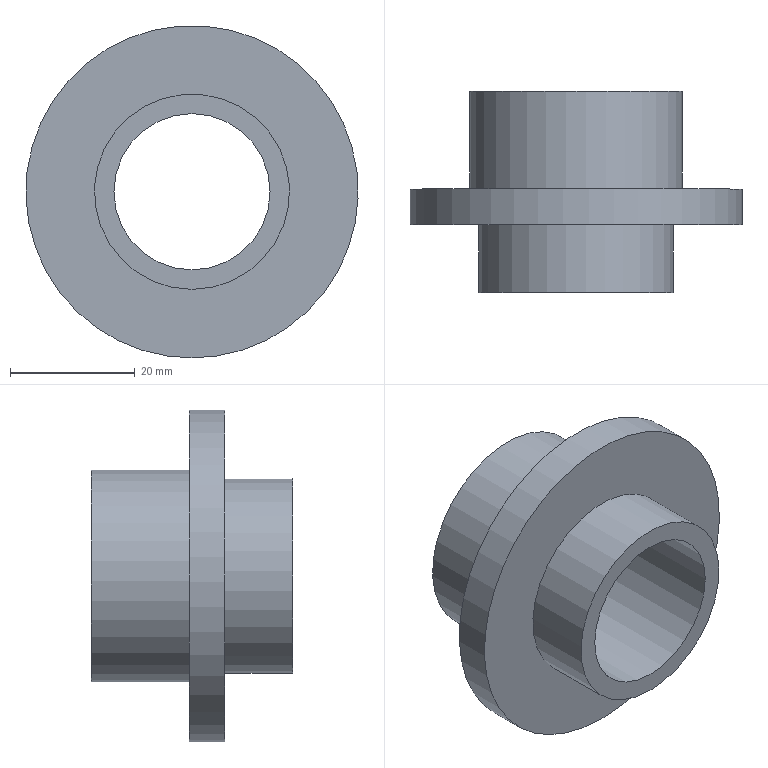Component | NX | SPRING_SLEEVE_1 | 1 solid | 8 faces | box 53.17 x 32.19 x 53.17 mm | volume 19347 mm3 | cylinder 4 | plane 4 | commonest cylinder face diameters 53.169 x1 31.237 x1 25 x1 34 x1
STEP:
#1=CARTESIAN_POINT('',(0.,0.,0.));
#2=DIRECTION('',(0.,0.,1.));
#3=DIRECTION('',(1.,0.,0.));
#4=AXIS2_PLACEMENT_3D('',#1,#2,#3);
#5=CARTESIAN_POINT('',(0.,0.,-26.584));
#6=VERTEX_POINT('',#5);
#7=CARTESIAN_POINT('',(0.,0.,0.));
#8=DIRECTION('',(0.,-1.,0.));
#9=DIRECTION('',(0.,0.,-1.));
#10=AXIS2_PLACEMENT_3D('',#7,#8,#9);
#11=CIRCLE('',#10,26.584);
#12=CARTESIAN_POINT('',(0.,0.,0.));
#13=DIRECTION('',(0.,-1.,0.));
#14=DIRECTION('',(0.,0.,-1.));
#15=AXIS2_PLACEMENT_3D('',#12,#13,#14);
#16=CYLINDRICAL_SURFACE('',#15,26.584);
#17=CARTESIAN_POINT('',(0.,-0.));
#18=DIRECTION('',(1.,0.));
#19=VECTOR('',#18,1.);
#20=LINE('',#17,#19);
#21=(GEOMETRIC_REPRESENTATION_CONTEXT(2)PARAMETRIC_REPRESENTATION_CONTEXT()REPRESENTATION_CONTEXT('',''));
#22=DEFINITIONAL_REPRESENTATION('',(#20),#21);
#23=PCURVE('',#16,#22);
#24=CARTESIAN_POINT('',(-26.584,0.,0.));
#25=DIRECTION('',(0.,1.,0.));
#26=DIRECTION('',(0.,0.,1.));
#27=AXIS2_PLACEMENT_3D('',#24,#25,#26);
#28=PLANE('',#27);
#29=CARTESIAN_POINT('',(-26.584,26.584));
#30=CARTESIAN_POINT('',(-26.584,72.63));
#31=CARTESIAN_POINT('',(13.292,49.607));
#32=CARTESIAN_POINT('',(53.169,26.584));
#33=CARTESIAN_POINT('',(13.292,3.562));
#34=CARTESIAN_POINT('',(-26.584,-19.461));
#35=CARTESIAN_POINT('',(-26.584,26.584));
#36=(BOUNDED_CURVE()B_SPLINE_CURVE(2,(#29,#30,#31,#32,#33,#34,#35),.UNSPECIFIED.,.T.,.F.)B_SPLINE_CURVE_WITH_KNOTS((1,2,2,2,2,1),(-2.094,0.,2.094,4.189,6.283,8.378),.UNSPECIFIED.)CURVE()GEOMETRIC_REPRESENTATION_ITEM()RATIONAL_B_SPLINE_CURVE((1.,0.5,1.,0.5,1.,0.5,1.))REPRESENTATION_ITEM(''));
#37=(GEOMETRIC_REPRESENTATION_CONTEXT(2)PARAMETRIC_REPRESENTATION_CONTEXT()REPRESENTATION_CONTEXT('',''));
#38=DEFINITIONAL_REPRESENTATION('',(#36),#37);
#39=PCURVE('',#28,#38);
#40=SURFACE_CURVE('',#11,(#23,#39),.PCURVE_S1.);
#41=EDGE_CURVE('',#6,#6,#40,.T.);
#42=ORIENTED_EDGE('',*,*,#41,.F.);
#43=CARTESIAN_POINT('',(0.,5.684,-26.584));
#44=VERTEX_POINT('',#43);
#45=CARTESIAN_POINT('',(-0.,5.684,-26.584));
#46=CARTESIAN_POINT('',(-0.,0.,-26.584));
#47=B_SPLINE_CURVE_WITH_KNOTS('',1,(#45,#46),.UNSPECIFIED.,.F.,.F.,(2,2),(-5.684,-0.),.PIECEWISE_BEZIER_KNOTS.);
#48=CARTESIAN_POINT('',(0.,0.));
#49=DIRECTION('',(0.,1.));
#50=VECTOR('',#49,1.);
#51=LINE('',#48,#50);
#52=(GEOMETRIC_REPRESENTATION_CONTEXT(2)PARAMETRIC_REPRESENTATION_CONTEXT()REPRESENTATION_CONTEXT('',''));
#53=DEFINITIONAL_REPRESENTATION('',(#51),#52);
#54=PCURVE('',#16,#53);
#55=CARTESIAN_POINT('',(6.283,0.));
#56=DIRECTION('',(0.,1.));
#57=VECTOR('',#56,1.);
#58=LINE('',#55,#57);
#59=(GEOMETRIC_REPRESENTATION_CONTEXT(2)PARAMETRIC_REPRESENTATION_CONTEXT()REPRESENTATION_CONTEXT('',''));
#60=DEFINITIONAL_REPRESENTATION('',(#58),#59);
#61=PCURVE('',#16,#60);
#62=SEAM_CURVE('',#47,(#54,#61),.PCURVE_S1.);
#63=EDGE_CURVE('',#44,#6,#62,.T.);
#64=ORIENTED_EDGE('',*,*,#63,.F.);
#65=CARTESIAN_POINT('',(0.,5.684,0.));
#66=DIRECTION('',(0.,-1.,0.));
#67=DIRECTION('',(0.,0.,-1.));
#68=AXIS2_PLACEMENT_3D('',#65,#66,#67);
#69=CIRCLE('',#68,26.584);
#70=CARTESIAN_POINT('',(0.,-5.684));
#71=DIRECTION('',(1.,0.));
#72=VECTOR('',#71,1.);
#73=LINE('',#70,#72);
#74=(GEOMETRIC_REPRESENTATION_CONTEXT(2)PARAMETRIC_REPRESENTATION_CONTEXT()REPRESENTATION_CONTEXT('',''));
#75=DEFINITIONAL_REPRESENTATION('',(#73),#74);
#76=PCURVE('',#16,#75);
#77=CARTESIAN_POINT('',(-17.456,5.684,0.));
#78=DIRECTION('',(0.,-1.,0.));
#79=DIRECTION('',(0.,0.,-1.));
#80=AXIS2_PLACEMENT_3D('',#77,#78,#79);
#81=PLANE('',#80);
#82=CARTESIAN_POINT('',(0.,17.456));
#83=DIRECTION('',(1.,0.));
#84=AXIS2_PLACEMENT_2D('',#82,#83);
#85=CIRCLE('',#84,26.584);
#86=(GEOMETRIC_REPRESENTATION_CONTEXT(2)PARAMETRIC_REPRESENTATION_CONTEXT()REPRESENTATION_CONTEXT('',''));
#87=DEFINITIONAL_REPRESENTATION('',(#85),#86);
#88=PCURVE('',#81,#87);
#89=SURFACE_CURVE('',#69,(#76,#88),.PCURVE_S1.);
#90=EDGE_CURVE('',#44,#44,#89,.T.);
#91=ORIENTED_EDGE('',*,*,#90,.T.);
#92=ORIENTED_EDGE('',*,*,#63,.T.);
#93=EDGE_LOOP('',(#42,#64,#91,#92));
#94=FACE_BOUND('',#93,.T.);
#95=ADVANCED_FACE('',(#94),#16,.T.);
#96=CARTESIAN_POINT('',(0.,0.,-15.619));
#97=VERTEX_POINT('',#96);
#98=CARTESIAN_POINT('',(0.,0.,0.));
#99=DIRECTION('',(0.,-1.,0.));
#100=DIRECTION('',(0.,0.,-1.));
#101=AXIS2_PLACEMENT_3D('',#98,#99,#100);
#102=CIRCLE('',#101,15.619);
#103=CARTESIAN_POINT('',(-15.619,26.584));
#104=CARTESIAN_POINT('',(-15.619,53.637));
#105=CARTESIAN_POINT('',(7.809,40.111));
#106=CARTESIAN_POINT('',(31.237,26.584));
#107=CARTESIAN_POINT('',(7.809,13.058));
#108=CARTESIAN_POINT('',(-15.619,-0.4679));
#109=CARTESIAN_POINT('',(-15.619,26.584));
#110=(BOUNDED_CURVE()B_SPLINE_CURVE(2,(#103,#104,#105,#106,#107,#108,#109),.UNSPECIFIED.,.T.,.F.)B_SPLINE_CURVE_WITH_KNOTS((1,2,2,2,2,1),(-2.094,0.,2.094,4.189,6.283,8.378),.UNSPECIFIED.)CURVE()GEOMETRIC_REPRESENTATION_ITEM()RATIONAL_B_SPLINE_CURVE((1.,0.5,1.,0.5,1.,0.5,1.))REPRESENTATION_ITEM(''));
#111=(GEOMETRIC_REPRESENTATION_CONTEXT(2)PARAMETRIC_REPRESENTATION_CONTEXT()REPRESENTATION_CONTEXT('',''));
#112=DEFINITIONAL_REPRESENTATION('',(#110),#111);
#113=PCURVE('',#28,#112);
#114=CARTESIAN_POINT('',(0.,0.,0.));
#115=DIRECTION('',(0.,-1.,0.));
#116=DIRECTION('',(0.,0.,-1.));
#117=AXIS2_PLACEMENT_3D('',#114,#115,#116);
#118=CYLINDRICAL_SURFACE('',#117,15.619);
#119=CARTESIAN_POINT('',(0.,0.));
#120=DIRECTION('',(1.,0.));
#121=VECTOR('',#120,1.);
#122=LINE('',#119,#121);
#123=(GEOMETRIC_REPRESENTATION_CONTEXT(2)PARAMETRIC_REPRESENTATION_CONTEXT()REPRESENTATION_CONTEXT('',''));
#124=DEFINITIONAL_REPRESENTATION('',(#122),#123);
#125=PCURVE('',#118,#124);
#126=SURFACE_CURVE('',#102,(#113,#125),.PCURVE_S1.);
#127=EDGE_CURVE('',#97,#97,#126,.T.);
#128=ORIENTED_EDGE('',*,*,#127,.F.);
#129=EDGE_LOOP('',(#128));
#130=FACE_BOUND('',#129,.T.);
#131=ORIENTED_EDGE('',*,*,#41,.T.);
#132=EDGE_LOOP('',(#131));
#133=FACE_BOUND('',#132,.T.);
#134=ADVANCED_FACE('',(#130,#133),#28,.F.);
#135=CARTESIAN_POINT('',(0.,-10.877,-15.619));
#136=VERTEX_POINT('',#135);
#137=CARTESIAN_POINT('',(0.,-10.877,0.));
#138=DIRECTION('',(0.,-1.,0.));
#139=DIRECTION('',(0.,0.,-1.));
#140=AXIS2_PLACEMENT_3D('',#137,#138,#139);
#141=CIRCLE('',#140,15.619);
#142=CARTESIAN_POINT('',(0.,10.877));
#143=DIRECTION('',(1.,0.));
#144=VECTOR('',#143,1.);
#145=LINE('',#142,#144);
#146=(GEOMETRIC_REPRESENTATION_CONTEXT(2)PARAMETRIC_REPRESENTATION_CONTEXT()REPRESENTATION_CONTEXT('',''));
#147=DEFINITIONAL_REPRESENTATION('',(#145),#146);
#148=PCURVE('',#118,#147);
#149=CARTESIAN_POINT('',(-15.619,-10.877,0.));
#150=DIRECTION('',(0.,1.,0.));
#151=DIRECTION('',(0.,0.,1.));
#152=AXIS2_PLACEMENT_3D('',#149,#150,#151);
#153=PLANE('',#152);
#154=CARTESIAN_POINT('',(-15.619,15.619));
#155=CARTESIAN_POINT('',(-15.619,42.671));
#156=CARTESIAN_POINT('',(7.809,29.145));
#157=CARTESIAN_POINT('',(31.237,15.619));
#158=CARTESIAN_POINT('',(7.809,2.093));
#159=CARTESIAN_POINT('',(-15.619,-11.434));
#160=CARTESIAN_POINT('',(-15.619,15.619));
#161=(BOUNDED_CURVE()B_SPLINE_CURVE(2,(#154,#155,#156,#157,#158,#159,#160),.UNSPECIFIED.,.T.,.F.)B_SPLINE_CURVE_WITH_KNOTS((1,2,2,2,2,1),(-2.094,0.,2.094,4.189,6.283,8.378),.UNSPECIFIED.)CURVE()GEOMETRIC_REPRESENTATION_ITEM()RATIONAL_B_SPLINE_CURVE((1.,0.5,1.,0.5,1.,0.5,1.))REPRESENTATION_ITEM(''));
#162=(GEOMETRIC_REPRESENTATION_CONTEXT(2)PARAMETRIC_REPRESENTATION_CONTEXT()REPRESENTATION_CONTEXT('',''));
#163=DEFINITIONAL_REPRESENTATION('',(#161),#162);
#164=PCURVE('',#153,#163);
#165=SURFACE_CURVE('',#141,(#148,#164),.PCURVE_S1.);
#166=EDGE_CURVE('',#136,#136,#165,.T.);
#167=ORIENTED_EDGE('',*,*,#166,.F.);
#168=CARTESIAN_POINT('',(-0.,0.,-15.619));
#169=CARTESIAN_POINT('',(-0.,-10.877,-15.619));
#170=B_SPLINE_CURVE_WITH_KNOTS('',1,(#168,#169),.UNSPECIFIED.,.F.,.F.,(2,2),(0.,10.877),.PIECEWISE_BEZIER_KNOTS.);
#171=CARTESIAN_POINT('',(0.,0.));
#172=DIRECTION('',(0.,1.));
#173=VECTOR('',#172,1.);
#174=LINE('',#171,#173);
#175=(GEOMETRIC_REPRESENTATION_CONTEXT(2)PARAMETRIC_REPRESENTATION_CONTEXT()REPRESENTATION_CONTEXT('',''));
#176=DEFINITIONAL_REPRESENTATION('',(#174),#175);
#177=PCURVE('',#118,#176);
#178=CARTESIAN_POINT('',(6.283,0.));
#179=DIRECTION('',(0.,1.));
#180=VECTOR('',#179,1.);
#181=LINE('',#178,#180);
#182=(GEOMETRIC_REPRESENTATION_CONTEXT(2)PARAMETRIC_REPRESENTATION_CONTEXT()REPRESENTATION_CONTEXT('',''));
#183=DEFINITIONAL_REPRESENTATION('',(#181),#182);
#184=PCURVE('',#118,#183);
#185=SEAM_CURVE('',#170,(#177,#184),.PCURVE_S1.);
#186=EDGE_CURVE('',#97,#136,#185,.T.);
#187=ORIENTED_EDGE('',*,*,#186,.F.);
#188=ORIENTED_EDGE('',*,*,#127,.T.);
#189=ORIENTED_EDGE('',*,*,#186,.T.);
#190=EDGE_LOOP('',(#167,#187,#188,#189));
#191=FACE_BOUND('',#190,.T.);
#192=ADVANCED_FACE('',(#191),#118,.T.);
#193=CARTESIAN_POINT('',(0.,-10.877,-12.5));
#194=VERTEX_POINT('',#193);
#195=CARTESIAN_POINT('',(0.,-10.877,0.));
#196=DIRECTION('',(0.,-1.,0.));
#197=DIRECTION('',(0.,0.,-1.));
#198=AXIS2_PLACEMENT_3D('',#195,#196,#197);
#199=CIRCLE('',#198,12.5);
#200=CARTESIAN_POINT('',(-12.5,15.619));
#201=CARTESIAN_POINT('',(-12.5,37.269));
#202=CARTESIAN_POINT('',(6.25,26.444));
#203=CARTESIAN_POINT('',(25.,15.619));
#204=CARTESIAN_POINT('',(6.25,4.793));
#205=CARTESIAN_POINT('',(-12.5,-6.032));
#206=CARTESIAN_POINT('',(-12.5,15.619));
#207=(BOUNDED_CURVE()B_SPLINE_CURVE(2,(#200,#201,#202,#203,#204,#205,#206),.UNSPECIFIED.,.T.,.F.)B_SPLINE_CURVE_WITH_KNOTS((1,2,2,2,2,1),(-2.094,0.,2.094,4.189,6.283,8.378),.UNSPECIFIED.)CURVE()GEOMETRIC_REPRESENTATION_ITEM()RATIONAL_B_SPLINE_CURVE((1.,0.5,1.,0.5,1.,0.5,1.))REPRESENTATION_ITEM(''));
#208=(GEOMETRIC_REPRESENTATION_CONTEXT(2)PARAMETRIC_REPRESENTATION_CONTEXT()REPRESENTATION_CONTEXT('',''));
#209=DEFINITIONAL_REPRESENTATION('',(#207),#208);
#210=PCURVE('',#153,#209);
#211=CARTESIAN_POINT('',(0.,0.,0.));
#212=DIRECTION('',(0.,-1.,0.));
#213=DIRECTION('',(0.,0.,-1.));
#214=AXIS2_PLACEMENT_3D('',#211,#212,#213);
#215=CYLINDRICAL_SURFACE('',#214,12.5);
#216=CARTESIAN_POINT('',(0.,10.877));
#217=DIRECTION('',(1.,0.));
#218=VECTOR('',#217,1.);
#219=LINE('',#216,#218);
#220=(GEOMETRIC_REPRESENTATION_CONTEXT(2)PARAMETRIC_REPRESENTATION_CONTEXT()REPRESENTATION_CONTEXT('',''));
#221=DEFINITIONAL_REPRESENTATION('',(#219),#220);
#222=PCURVE('',#215,#221);
#223=SURFACE_CURVE('',#199,(#210,#222),.PCURVE_S1.);
#224=EDGE_CURVE('',#194,#194,#223,.T.);
#225=ORIENTED_EDGE('',*,*,#224,.F.);
#226=EDGE_LOOP('',(#225));
#227=FACE_BOUND('',#226,.T.);
#228=ORIENTED_EDGE('',*,*,#166,.T.);
#229=EDGE_LOOP('',(#228));
#230=FACE_BOUND('',#229,.T.);
#231=ADVANCED_FACE('',(#227,#230),#153,.F.);
#232=CARTESIAN_POINT('',(0.,21.318,-12.5));
#233=VERTEX_POINT('',#232);
#234=CARTESIAN_POINT('',(0.,21.318,0.));
#235=DIRECTION('',(0.,-1.,0.));
#236=DIRECTION('',(0.,0.,-1.));
#237=AXIS2_PLACEMENT_3D('',#234,#235,#236);
#238=CIRCLE('',#237,12.5);
#239=CARTESIAN_POINT('',(0.,-21.318));
#240=DIRECTION('',(1.,0.));
#241=VECTOR('',#240,1.);
#242=LINE('',#239,#241);
#243=(GEOMETRIC_REPRESENTATION_CONTEXT(2)PARAMETRIC_REPRESENTATION_CONTEXT()REPRESENTATION_CONTEXT('',''));
#244=DEFINITIONAL_REPRESENTATION('',(#242),#243);
#245=PCURVE('',#215,#244);
#246=CARTESIAN_POINT('',(-12.5,21.318,0.));
#247=DIRECTION('',(0.,-1.,0.));
#248=DIRECTION('',(0.,0.,-1.));
#249=AXIS2_PLACEMENT_3D('',#246,#247,#248);
#250=PLANE('',#249);
#251=CARTESIAN_POINT('',(0.,12.5));
#252=DIRECTION('',(1.,0.));
#253=AXIS2_PLACEMENT_2D('',#251,#252);
#254=CIRCLE('',#253,12.5);
#255=(GEOMETRIC_REPRESENTATION_CONTEXT(2)PARAMETRIC_REPRESENTATION_CONTEXT()REPRESENTATION_CONTEXT('',''));
#256=DEFINITIONAL_REPRESENTATION('',(#254),#255);
#257=PCURVE('',#250,#256);
#258=SURFACE_CURVE('',#238,(#245,#257),.PCURVE_S1.);
#259=EDGE_CURVE('',#233,#233,#258,.T.);
#260=ORIENTED_EDGE('',*,*,#259,.T.);
#261=CARTESIAN_POINT('',(0.,21.318,-12.5));
#262=CARTESIAN_POINT('',(0.,-10.877,-12.5));
#263=B_SPLINE_CURVE_WITH_KNOTS('',1,(#261,#262),.UNSPECIFIED.,.F.,.F.,(2,2),(-21.318,10.877),.PIECEWISE_BEZIER_KNOTS.);
#264=CARTESIAN_POINT('',(6.283,0.));
#265=DIRECTION('',(0.,1.));
#266=VECTOR('',#265,1.);
#267=LINE('',#264,#266);
#268=(GEOMETRIC_REPRESENTATION_CONTEXT(2)PARAMETRIC_REPRESENTATION_CONTEXT()REPRESENTATION_CONTEXT('',''));
#269=DEFINITIONAL_REPRESENTATION('',(#267),#268);
#270=PCURVE('',#215,#269);
#271=CARTESIAN_POINT('',(0.,0.));
#272=DIRECTION('',(0.,1.));
#273=VECTOR('',#272,1.);
#274=LINE('',#271,#273);
#275=(GEOMETRIC_REPRESENTATION_CONTEXT(2)PARAMETRIC_REPRESENTATION_CONTEXT()REPRESENTATION_CONTEXT('',''));
#276=DEFINITIONAL_REPRESENTATION('',(#274),#275);
#277=PCURVE('',#215,#276);
#278=SEAM_CURVE('',#263,(#270,#277),.PCURVE_S1.);
#279=EDGE_CURVE('',#233,#194,#278,.T.);
#280=ORIENTED_EDGE('',*,*,#279,.T.);
#281=ORIENTED_EDGE('',*,*,#224,.F.);
#282=ORIENTED_EDGE('',*,*,#279,.F.);
#283=EDGE_LOOP('',(#260,#280,#281,#282));
#284=FACE_BOUND('',#283,.F.);
#285=ADVANCED_FACE('',(#284),#215,.F.);
#286=CARTESIAN_POINT('',(0.,21.318,-17.));
#287=VERTEX_POINT('',#286);
#288=CARTESIAN_POINT('',(0.,21.318,0.));
#289=DIRECTION('',(0.,-1.,0.));
#290=DIRECTION('',(0.,0.,-1.));
#291=AXIS2_PLACEMENT_3D('',#288,#289,#290);
#292=CIRCLE('',#291,17.);
#293=CARTESIAN_POINT('',(0.,12.5));
#294=DIRECTION('',(1.,0.));
#295=AXIS2_PLACEMENT_2D('',#293,#294);
#296=CIRCLE('',#295,17.);
#297=(GEOMETRIC_REPRESENTATION_CONTEXT(2)PARAMETRIC_REPRESENTATION_CONTEXT()REPRESENTATION_CONTEXT('',''));
#298=DEFINITIONAL_REPRESENTATION('',(#296),#297);
#299=PCURVE('',#250,#298);
#300=CARTESIAN_POINT('',(0.,0.,0.));
#301=DIRECTION('',(0.,-1.,0.));
#302=DIRECTION('',(0.,0.,-1.));
#303=AXIS2_PLACEMENT_3D('',#300,#301,#302);
#304=CYLINDRICAL_SURFACE('',#303,17.);
#305=CARTESIAN_POINT('',(0.,-21.318));
#306=DIRECTION('',(1.,0.));
#307=VECTOR('',#306,1.);
#308=LINE('',#305,#307);
#309=(GEOMETRIC_REPRESENTATION_CONTEXT(2)PARAMETRIC_REPRESENTATION_CONTEXT()REPRESENTATION_CONTEXT('',''));
#310=DEFINITIONAL_REPRESENTATION('',(#308),#309);
#311=PCURVE('',#304,#310);
#312=SURFACE_CURVE('',#292,(#299,#311),.PCURVE_S1.);
#313=EDGE_CURVE('',#287,#287,#312,.T.);
#314=ORIENTED_EDGE('',*,*,#313,.F.);
#315=EDGE_LOOP('',(#314));
#316=FACE_BOUND('',#315,.T.);
#317=ORIENTED_EDGE('',*,*,#259,.T.);
#318=EDGE_LOOP('',(#317));
#319=FACE_BOUND('',#318,.T.);
#320=ADVANCED_FACE('',(#316,#319),#250,.F.);
#321=CARTESIAN_POINT('',(0.,5.684,-17.));
#322=VERTEX_POINT('',#321);
#323=CARTESIAN_POINT('',(0.,5.684,0.));
#324=DIRECTION('',(0.,-1.,0.));
#325=DIRECTION('',(0.,0.,-1.));
#326=AXIS2_PLACEMENT_3D('',#323,#324,#325);
#327=CIRCLE('',#326,17.);
#328=CARTESIAN_POINT('',(0.,-5.684));
#329=DIRECTION('',(1.,0.));
#330=VECTOR('',#329,1.);
#331=LINE('',#328,#330);
#332=(GEOMETRIC_REPRESENTATION_CONTEXT(2)PARAMETRIC_REPRESENTATION_CONTEXT()REPRESENTATION_CONTEXT('',''));
#333=DEFINITIONAL_REPRESENTATION('',(#331),#332);
#334=PCURVE('',#304,#333);
#335=CARTESIAN_POINT('',(0.,17.456));
#336=DIRECTION('',(1.,0.));
#337=AXIS2_PLACEMENT_2D('',#335,#336);
#338=CIRCLE('',#337,17.);
#339=(GEOMETRIC_REPRESENTATION_CONTEXT(2)PARAMETRIC_REPRESENTATION_CONTEXT()REPRESENTATION_CONTEXT('',''));
#340=DEFINITIONAL_REPRESENTATION('',(#338),#339);
#341=PCURVE('',#81,#340);
#342=SURFACE_CURVE('',#327,(#334,#341),.PCURVE_S1.);
#343=EDGE_CURVE('',#322,#322,#342,.T.);
#344=ORIENTED_EDGE('',*,*,#343,.F.);
#345=CARTESIAN_POINT('',(-0.,21.318,-17.));
#346=CARTESIAN_POINT('',(-0.,5.684,-17.));
#347=B_SPLINE_CURVE_WITH_KNOTS('',1,(#345,#346),.UNSPECIFIED.,.F.,.F.,(2,2),(-21.318,-5.684),.PIECEWISE_BEZIER_KNOTS.);
#348=CARTESIAN_POINT('',(0.,0.));
#349=DIRECTION('',(0.,1.));
#350=VECTOR('',#349,1.);
#351=LINE('',#348,#350);
#352=(GEOMETRIC_REPRESENTATION_CONTEXT(2)PARAMETRIC_REPRESENTATION_CONTEXT()REPRESENTATION_CONTEXT('',''));
#353=DEFINITIONAL_REPRESENTATION('',(#351),#352);
#354=PCURVE('',#304,#353);
#355=CARTESIAN_POINT('',(6.283,0.));
#356=DIRECTION('',(0.,1.));
#357=VECTOR('',#356,1.);
#358=LINE('',#355,#357);
#359=(GEOMETRIC_REPRESENTATION_CONTEXT(2)PARAMETRIC_REPRESENTATION_CONTEXT()REPRESENTATION_CONTEXT('',''));
#360=DEFINITIONAL_REPRESENTATION('',(#358),#359);
#361=PCURVE('',#304,#360);
#362=SEAM_CURVE('',#347,(#354,#361),.PCURVE_S1.);
#363=EDGE_CURVE('',#287,#322,#362,.T.);
#364=ORIENTED_EDGE('',*,*,#363,.F.);
#365=ORIENTED_EDGE('',*,*,#313,.T.);
#366=ORIENTED_EDGE('',*,*,#363,.T.);
#367=EDGE_LOOP('',(#344,#364,#365,#366));
#368=FACE_BOUND('',#367,.T.);
#369=ADVANCED_FACE('',(#368),#304,.T.);
#370=ORIENTED_EDGE('',*,*,#90,.F.);
#371=EDGE_LOOP('',(#370));
#372=FACE_BOUND('',#371,.T.);
#373=ORIENTED_EDGE('',*,*,#343,.T.);
#374=EDGE_LOOP('',(#373));
#375=FACE_BOUND('',#374,.T.);
#376=ADVANCED_FACE('',(#372,#375),#81,.F.);
#377=CLOSED_SHELL('',(#95,#134,#192,#231,#285,#320,#369,#376));
#378=MANIFOLD_SOLID_BREP('',#377);
#379=(LENGTH_UNIT()NAMED_UNIT(*)SI_UNIT(.MILLI.,.METRE.));
#380=UNCERTAINTY_MEASURE_WITH_UNIT(LENGTH_MEASURE(0.00001),#379,'','');
#381=(NAMED_UNIT(*)PLANE_ANGLE_UNIT()SI_UNIT($,.RADIAN.));
#382=(NAMED_UNIT(*)SI_UNIT($,.STERADIAN.)SOLID_ANGLE_UNIT());
#383=(GEOMETRIC_REPRESENTATION_CONTEXT(3)GLOBAL_UNCERTAINTY_ASSIGNED_CONTEXT((#380))GLOBAL_UNIT_ASSIGNED_CONTEXT((#379,#381,#382))REPRESENTATION_CONTEXT('',''));
#384=ADVANCED_BREP_SHAPE_REPRESENTATION('',(#4,#378),#383);